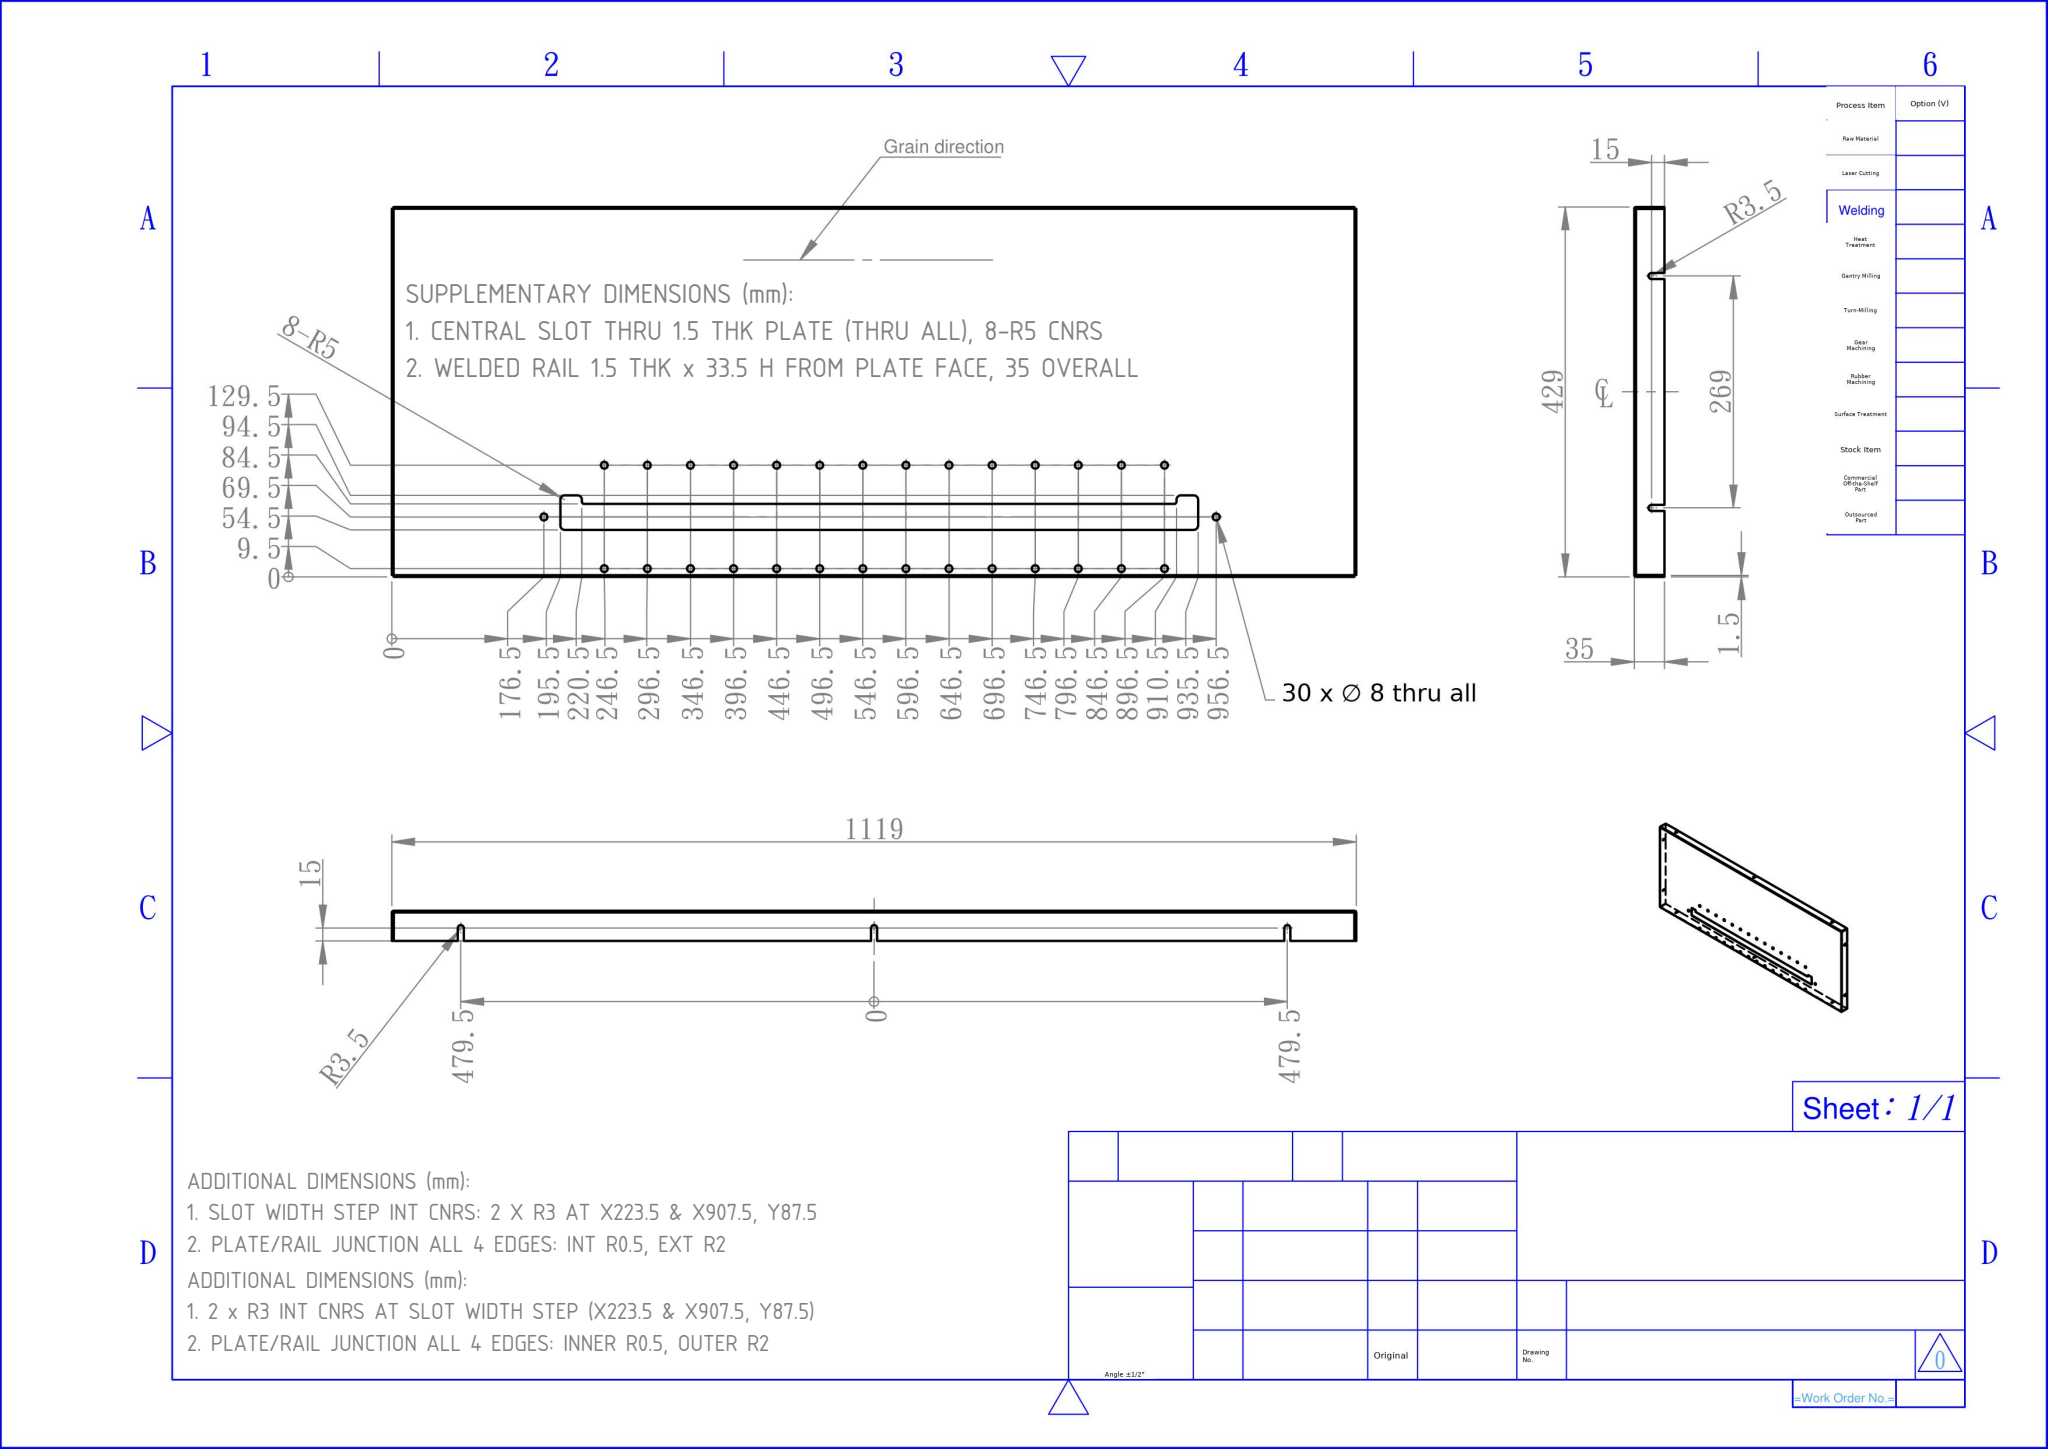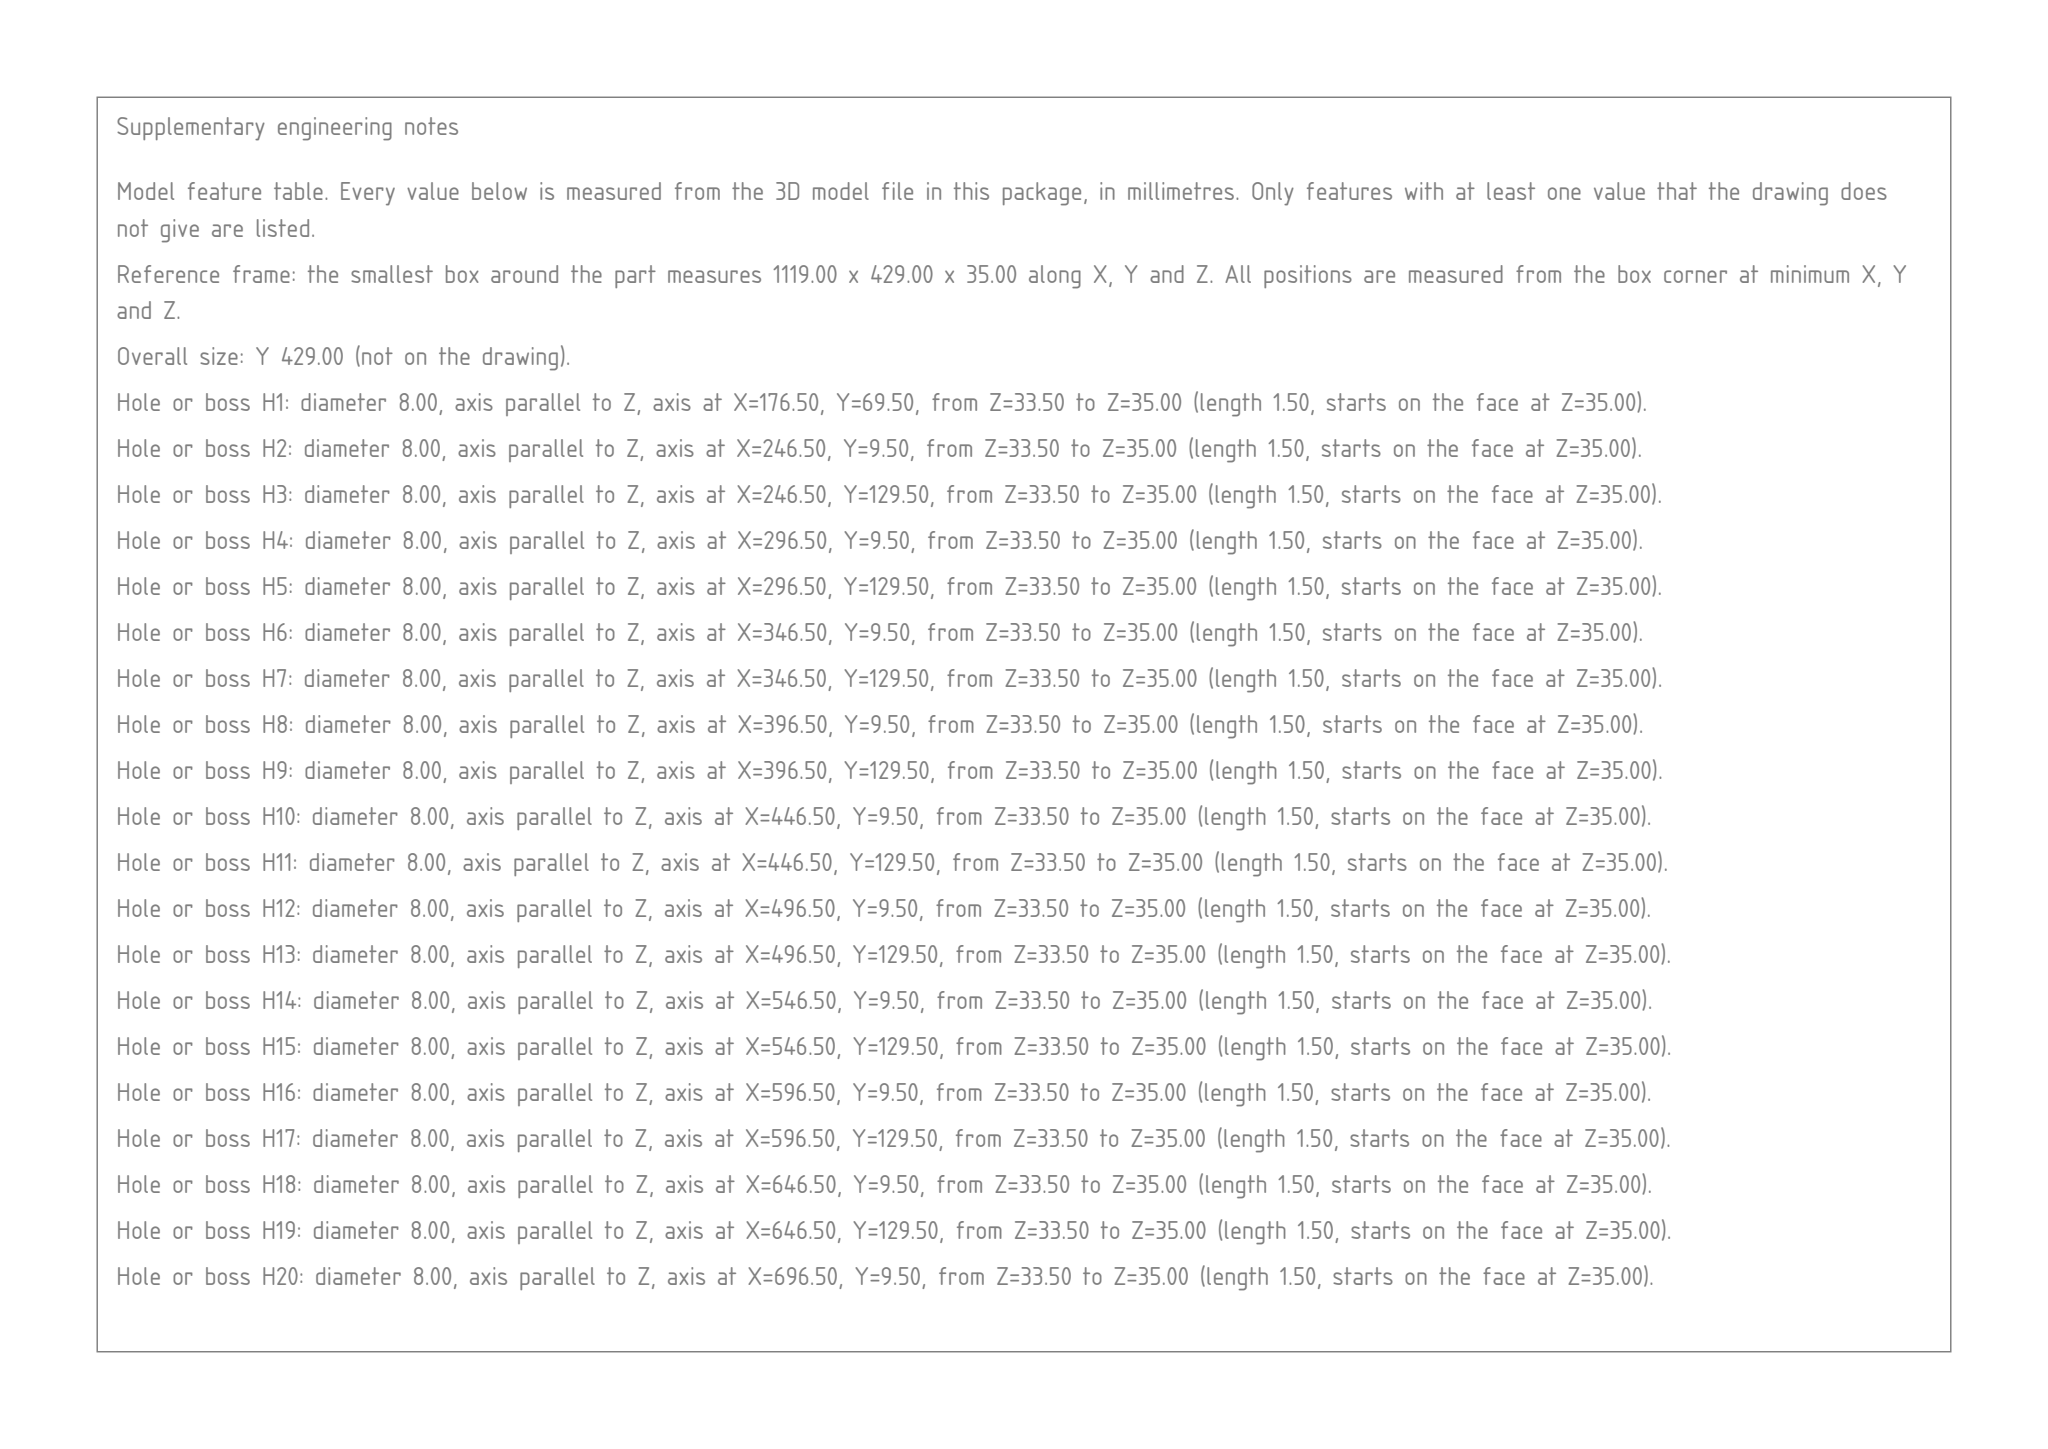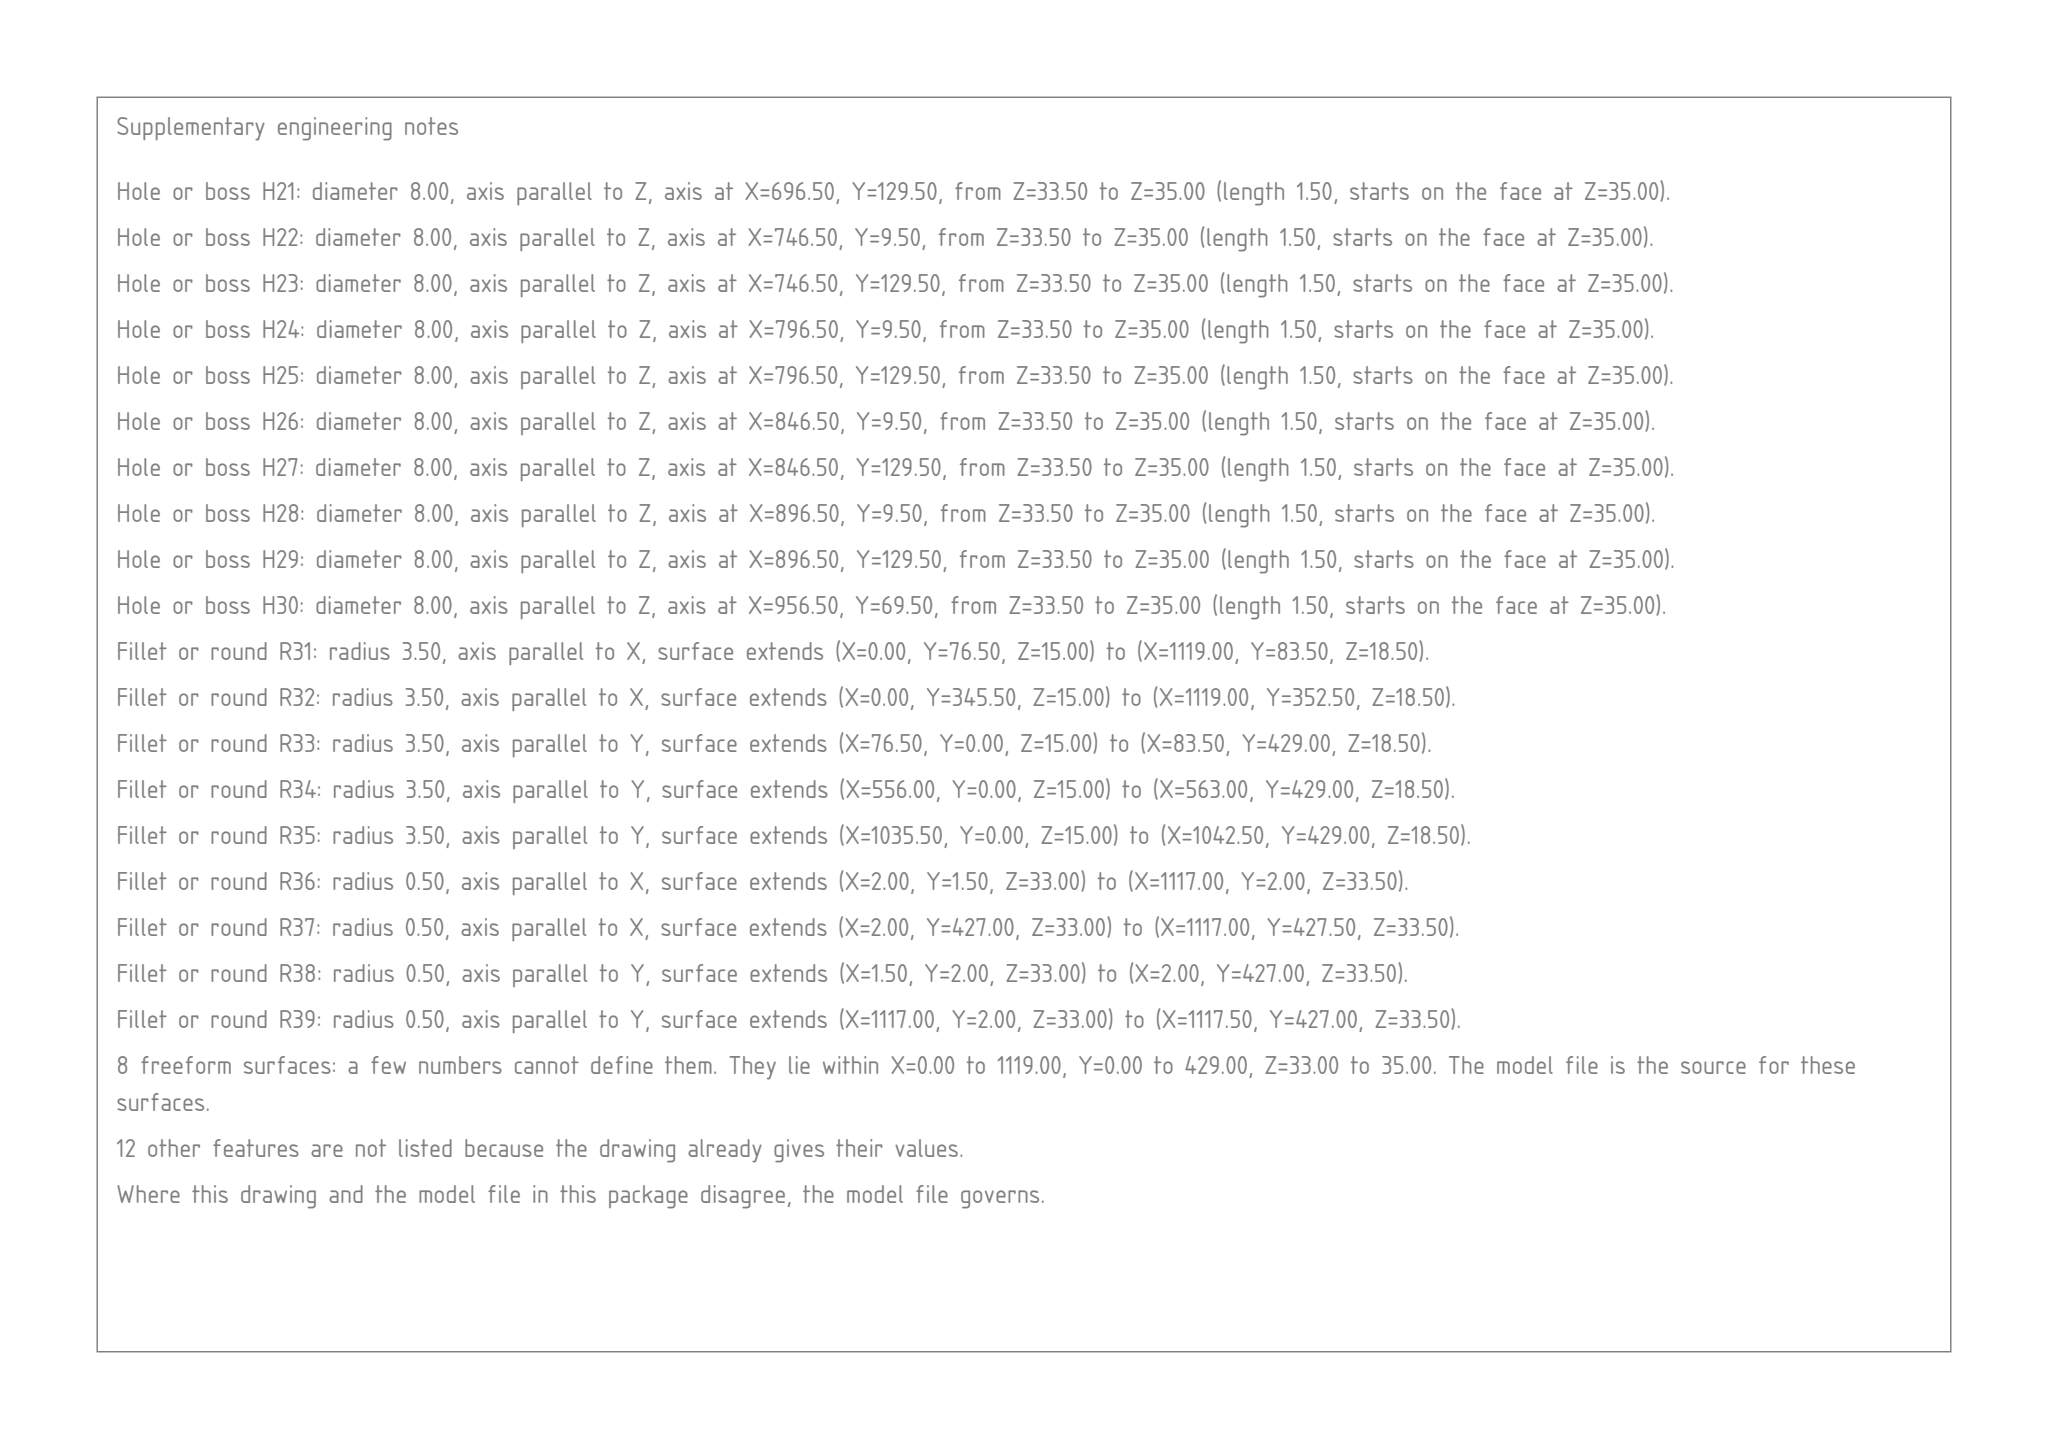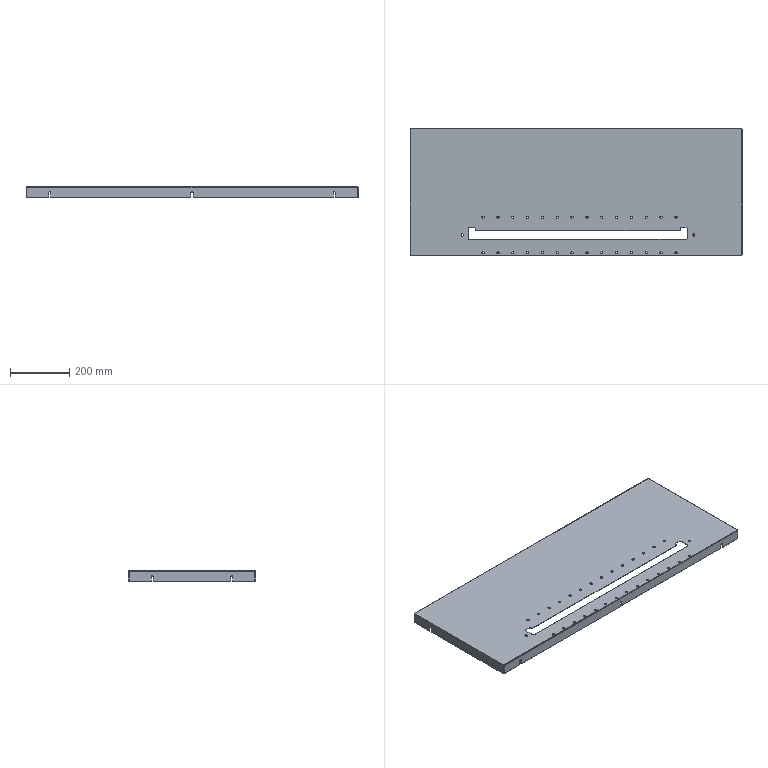Part | SolidWorks | mm | 1 solid | 160 faces | box 1119 x 429 x 35 mm | volume 834126 mm3 | cylinder 92 | plane 60 | spline 8 | commonest cylinder face diameters 8 x60 7 x16 10 x6 4 x4 1 x4 6 x2